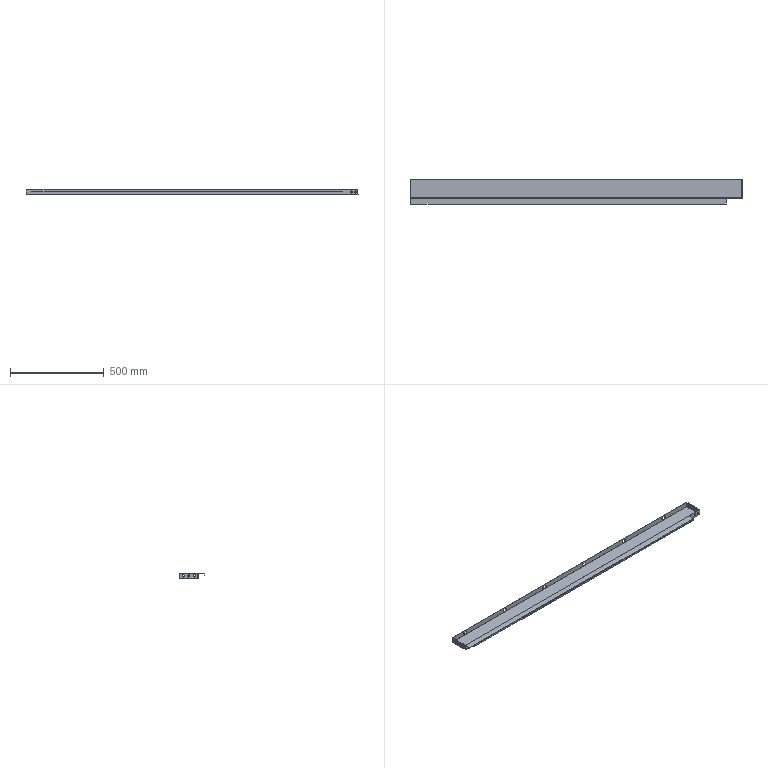Component | SolidWorks | UpperCrossbeam20001234-2 | 1 solid | 108 faces | volume 524373 mm3 | plane 62 | cylinder 46 | commonest cylinder face diameters 11 x34 3.4 x5 0.4 x5 7 x1 4 x1